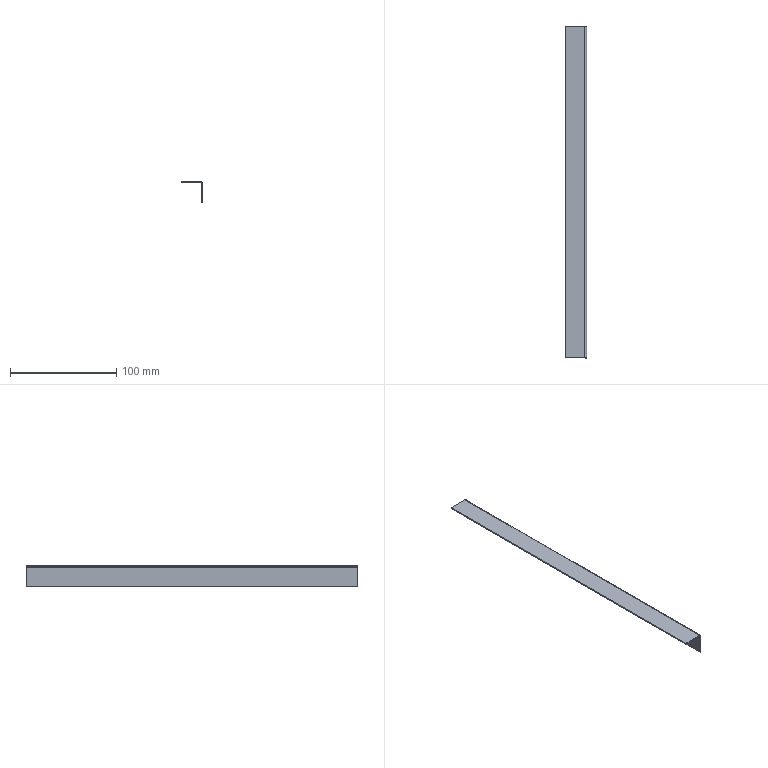Component | SolidWorks | CCQ-1.1-22VerticalAngleIron-1 | 1 solid | 14 faces | box 20 x 312 x 20 mm | volume 12002 mm3 | plane 12 | cylinder 2 | commonest cylinder face diameters 1.473 x1 3.473 x1 | material 304
STEP:
#1=COLOUR_RGB('',0.7922,0.8196,0.9333);
#2=FILL_AREA_STYLE_COLOUR('',#1);
#3=FILL_AREA_STYLE('',(#2));
#4=SURFACE_STYLE_FILL_AREA(#3);
#5=SURFACE_SIDE_STYLE('',(#4));
#6=SURFACE_STYLE_USAGE(.BOTH.,#5);
#7=PRESENTATION_STYLE_ASSIGNMENT((#6));
#8=CARTESIAN_POINT('',(0.6009,-4.902,-7.953));
#9=VERTEX_POINT('',#8);
#10=CARTESIAN_POINT('',(0.6009,-4.902,-7.992));
#11=VERTEX_POINT('',#10);
#12=CARTESIAN_POINT('',(0.6009,-4.902,-7.953));
#13=DIRECTION('',(-0.,0.,-1.));
#14=VECTOR('',#13,39.37);
#15=LINE('',#12,#14);
#16=EDGE_CURVE('',#9,#11,#15,.T.);
#17=ORIENTED_EDGE('',*,*,#16,.F.);
#18=CARTESIAN_POINT('',(0.6693,-4.902,-8.021));
#19=VERTEX_POINT('',#18);
#20=CARTESIAN_POINT('',(0.6009,-4.902,-8.021));
#21=DIRECTION('',(-0.,1.,0.));
#22=DIRECTION('',(0.,0.,1.));
#23=AXIS2_PLACEMENT_3D('',#20,#21,#22);
#24=CIRCLE('',#23,0.06837);
#25=EDGE_CURVE('',#9,#19,#24,.T.);
#26=ORIENTED_EDGE('',*,*,#25,.T.);
#27=CARTESIAN_POINT('',(0.6299,-4.902,-8.021));
#28=VERTEX_POINT('',#27);
#29=CARTESIAN_POINT('',(0.6299,-4.902,-8.021));
#30=DIRECTION('',(1.,0.,0.));
#31=VECTOR('',#30,39.37);
#32=LINE('',#29,#31);
#33=EDGE_CURVE('',#28,#19,#32,.T.);
#34=ORIENTED_EDGE('',*,*,#33,.F.);
#35=CARTESIAN_POINT('',(0.6009,-4.902,-8.021));
#36=DIRECTION('',(-0.,1.,0.));
#37=DIRECTION('',(-0.,0.,-1.));
#38=AXIS2_PLACEMENT_3D('',#35,#36,#37);
#39=CIRCLE('',#38,0.029);
#40=EDGE_CURVE('',#11,#28,#39,.T.);
#41=ORIENTED_EDGE('',*,*,#40,.F.);
#42=EDGE_LOOP('',(#17,#26,#34,#41));
#43=FACE_OUTER_BOUND('',#42,.T.);
#44=CARTESIAN_POINT('',(0.6009,-4.902,-7.953));
#45=DIRECTION('',(-0.,1.,0.));
#46=DIRECTION('',(-0.,0.,-1.));
#47=AXIS2_PLACEMENT_3D('',#44,#45,#46);
#48=PLANE('',#47);
#49=ADVANCED_FACE('',(#43),#48,.T.);
#50=CARTESIAN_POINT('',(-0.1181,-4.902,-7.953));
#51=VERTEX_POINT('',#50);
#52=CARTESIAN_POINT('',(-0.1181,-4.902,-7.953));
#53=DIRECTION('',(1.,0.,0.));
#54=VECTOR('',#53,39.37);
#55=LINE('',#52,#54);
#56=EDGE_CURVE('',#51,#9,#55,.T.);
#57=ORIENTED_EDGE('',*,*,#56,.T.);
#58=ORIENTED_EDGE('',*,*,#16,.T.);
#59=CARTESIAN_POINT('',(-0.1181,-4.902,-7.992));
#60=VERTEX_POINT('',#59);
#61=CARTESIAN_POINT('',(-0.1181,-4.902,-7.992));
#62=DIRECTION('',(1.,0.,0.));
#63=VECTOR('',#62,39.37);
#64=LINE('',#61,#63);
#65=EDGE_CURVE('',#60,#11,#64,.T.);
#66=ORIENTED_EDGE('',*,*,#65,.F.);
#67=CARTESIAN_POINT('',(-0.1181,-4.902,-7.953));
#68=DIRECTION('',(-0.,0.,-1.));
#69=VECTOR('',#68,39.37);
#70=LINE('',#67,#69);
#71=EDGE_CURVE('',#51,#60,#70,.T.);
#72=ORIENTED_EDGE('',*,*,#71,.F.);
#73=EDGE_LOOP('',(#57,#58,#66,#72));
#74=FACE_OUTER_BOUND('',#73,.T.);
#75=CARTESIAN_POINT('',(0.6299,-4.902,-8.021));
#76=DIRECTION('',(-0.,1.,0.));
#77=DIRECTION('',(-0.,0.,-1.));
#78=AXIS2_PLACEMENT_3D('',#75,#76,#77);
#79=PLANE('',#78);
#80=ADVANCED_FACE('',(#74),#79,.T.);
#81=CARTESIAN_POINT('',(0.6693,-17.185,-8.021));
#82=VERTEX_POINT('',#81);
#83=CARTESIAN_POINT('',(0.6299,-17.185,-8.021));
#84=VERTEX_POINT('',#83);
#85=CARTESIAN_POINT('',(0.6693,-17.185,-8.021));
#86=DIRECTION('',(-1.,-0.,-0.));
#87=VECTOR('',#86,39.37);
#88=LINE('',#85,#87);
#89=EDGE_CURVE('',#82,#84,#88,.T.);
#90=ORIENTED_EDGE('',*,*,#89,.F.);
#91=CARTESIAN_POINT('',(0.6009,-17.185,-7.953));
#92=VERTEX_POINT('',#91);
#93=CARTESIAN_POINT('',(0.6009,-17.185,-8.021));
#94=DIRECTION('',(-0.,1.,0.));
#95=DIRECTION('',(0.,0.,1.));
#96=AXIS2_PLACEMENT_3D('',#93,#94,#95);
#97=CIRCLE('',#96,0.06837);
#98=EDGE_CURVE('',#92,#82,#97,.T.);
#99=ORIENTED_EDGE('',*,*,#98,.F.);
#100=CARTESIAN_POINT('',(0.6009,-17.185,-7.992));
#101=VERTEX_POINT('',#100);
#102=CARTESIAN_POINT('',(0.6009,-17.185,-7.992));
#103=DIRECTION('',(0.,-0.,1.));
#104=VECTOR('',#103,39.37);
#105=LINE('',#102,#104);
#106=EDGE_CURVE('',#101,#92,#105,.T.);
#107=ORIENTED_EDGE('',*,*,#106,.F.);
#108=CARTESIAN_POINT('',(0.6009,-17.185,-8.021));
#109=DIRECTION('',(-0.,1.,0.));
#110=DIRECTION('',(-0.,0.,-1.));
#111=AXIS2_PLACEMENT_3D('',#108,#109,#110);
#112=CIRCLE('',#111,0.029);
#113=EDGE_CURVE('',#101,#84,#112,.T.);
#114=ORIENTED_EDGE('',*,*,#113,.T.);
#115=EDGE_LOOP('',(#90,#99,#107,#114));
#116=FACE_OUTER_BOUND('',#115,.T.);
#117=CARTESIAN_POINT('',(0.6693,-17.185,-8.021));
#118=DIRECTION('',(0.,-1.,-0.));
#119=DIRECTION('',(0.,-0.,1.));
#120=AXIS2_PLACEMENT_3D('',#117,#118,#119);
#121=PLANE('',#120);
#122=ADVANCED_FACE('',(#116),#121,.T.);
#123=CARTESIAN_POINT('',(0.6693,-17.185,-8.74));
#124=VERTEX_POINT('',#123);
#125=CARTESIAN_POINT('',(0.6693,-17.185,-7.953));
#126=DIRECTION('',(-0.,0.,-1.));
#127=VECTOR('',#126,39.37);
#128=LINE('',#125,#127);
#129=EDGE_CURVE('',#82,#124,#128,.T.);
#130=ORIENTED_EDGE('',*,*,#129,.F.);
#131=ORIENTED_EDGE('',*,*,#89,.T.);
#132=CARTESIAN_POINT('',(0.6299,-17.185,-8.74));
#133=VERTEX_POINT('',#132);
#134=CARTESIAN_POINT('',(0.6299,-17.185,-7.953));
#135=DIRECTION('',(-0.,0.,-1.));
#136=VECTOR('',#135,39.37);
#137=LINE('',#134,#136);
#138=EDGE_CURVE('',#84,#133,#137,.T.);
#139=ORIENTED_EDGE('',*,*,#138,.T.);
#140=CARTESIAN_POINT('',(0.6299,-17.185,-8.74));
#141=DIRECTION('',(1.,0.,0.));
#142=VECTOR('',#141,39.37);
#143=LINE('',#140,#142);
#144=EDGE_CURVE('',#133,#124,#143,.T.);
#145=ORIENTED_EDGE('',*,*,#144,.T.);
#146=EDGE_LOOP('',(#130,#131,#139,#145));
#147=FACE_OUTER_BOUND('',#146,.T.);
#148=CARTESIAN_POINT('',(0.6009,-17.185,-7.992));
#149=DIRECTION('',(0.,-1.,-0.));
#150=DIRECTION('',(0.,-0.,1.));
#151=AXIS2_PLACEMENT_3D('',#148,#149,#150);
#152=PLANE('',#151);
#153=ADVANCED_FACE('',(#147),#152,.T.);
#154=ORIENTED_EDGE('',*,*,#129,.T.);
#155=CARTESIAN_POINT('',(0.6693,-4.902,-8.74));
#156=VERTEX_POINT('',#155);
#157=CARTESIAN_POINT('',(0.6693,-4.902,-8.74));
#158=DIRECTION('',(0.,-1.,-0.));
#159=VECTOR('',#158,39.37);
#160=LINE('',#157,#159);
#161=EDGE_CURVE('',#156,#124,#160,.T.);
#162=ORIENTED_EDGE('',*,*,#161,.F.);
#163=CARTESIAN_POINT('',(0.6693,-4.902,-7.953));
#164=DIRECTION('',(-0.,0.,-1.));
#165=VECTOR('',#164,39.37);
#166=LINE('',#163,#165);
#167=EDGE_CURVE('',#19,#156,#166,.T.);
#168=ORIENTED_EDGE('',*,*,#167,.F.);
#169=CARTESIAN_POINT('',(0.6693,-4.902,-8.021));
#170=DIRECTION('',(0.,-1.,-0.));
#171=VECTOR('',#170,39.37);
#172=LINE('',#169,#171);
#173=EDGE_CURVE('',#19,#82,#172,.T.);
#174=ORIENTED_EDGE('',*,*,#173,.T.);
#175=EDGE_LOOP('',(#154,#162,#168,#174));
#176=FACE_OUTER_BOUND('',#175,.T.);
#177=CARTESIAN_POINT('',(0.6693,-4.902,-7.953));
#178=DIRECTION('',(-1.,-0.,-0.));
#179=DIRECTION('',(-0.,1.,0.));
#180=AXIS2_PLACEMENT_3D('',#177,#178,#179);
#181=PLANE('',#180);
#182=ADVANCED_FACE('',(#176),#181,.F.);
#183=ORIENTED_EDGE('',*,*,#144,.F.);
#184=CARTESIAN_POINT('',(0.6299,-4.902,-8.74));
#185=VERTEX_POINT('',#184);
#186=CARTESIAN_POINT('',(0.6299,-4.902,-8.74));
#187=DIRECTION('',(0.,-1.,-0.));
#188=VECTOR('',#187,39.37);
#189=LINE('',#186,#188);
#190=EDGE_CURVE('',#185,#133,#189,.T.);
#191=ORIENTED_EDGE('',*,*,#190,.F.);
#192=CARTESIAN_POINT('',(0.6299,-4.902,-8.74));
#193=DIRECTION('',(1.,0.,0.));
#194=VECTOR('',#193,39.37);
#195=LINE('',#192,#194);
#196=EDGE_CURVE('',#185,#156,#195,.T.);
#197=ORIENTED_EDGE('',*,*,#196,.T.);
#198=ORIENTED_EDGE('',*,*,#161,.T.);
#199=EDGE_LOOP('',(#183,#191,#197,#198));
#200=FACE_OUTER_BOUND('',#199,.T.);
#201=CARTESIAN_POINT('',(0.6299,-4.902,-8.74));
#202=DIRECTION('',(-0.,0.,-1.));
#203=DIRECTION('',(0.,-1.,-0.));
#204=AXIS2_PLACEMENT_3D('',#201,#202,#203);
#205=PLANE('',#204);
#206=ADVANCED_FACE('',(#200),#205,.T.);
#207=ORIENTED_EDGE('',*,*,#138,.F.);
#208=CARTESIAN_POINT('',(0.6299,-4.902,-8.021));
#209=DIRECTION('',(0.,-1.,-0.));
#210=VECTOR('',#209,39.37);
#211=LINE('',#208,#210);
#212=EDGE_CURVE('',#28,#84,#211,.T.);
#213=ORIENTED_EDGE('',*,*,#212,.F.);
#214=CARTESIAN_POINT('',(0.6299,-4.902,-7.953));
#215=DIRECTION('',(-0.,0.,-1.));
#216=VECTOR('',#215,39.37);
#217=LINE('',#214,#216);
#218=EDGE_CURVE('',#28,#185,#217,.T.);
#219=ORIENTED_EDGE('',*,*,#218,.T.);
#220=ORIENTED_EDGE('',*,*,#190,.T.);
#221=EDGE_LOOP('',(#207,#213,#219,#220));
#222=FACE_OUTER_BOUND('',#221,.T.);
#223=CARTESIAN_POINT('',(0.6299,-4.902,-7.953));
#224=DIRECTION('',(-1.,-0.,-0.));
#225=DIRECTION('',(-0.,1.,0.));
#226=AXIS2_PLACEMENT_3D('',#223,#224,#225);
#227=PLANE('',#226);
#228=ADVANCED_FACE('',(#222),#227,.T.);
#229=ORIENTED_EDGE('',*,*,#113,.F.);
#230=CARTESIAN_POINT('',(0.6009,-4.902,-7.992));
#231=DIRECTION('',(0.,-1.,-0.));
#232=VECTOR('',#231,39.37);
#233=LINE('',#230,#232);
#234=EDGE_CURVE('',#11,#101,#233,.T.);
#235=ORIENTED_EDGE('',*,*,#234,.F.);
#236=ORIENTED_EDGE('',*,*,#40,.T.);
#237=ORIENTED_EDGE('',*,*,#212,.T.);
#238=EDGE_LOOP('',(#229,#235,#236,#237));
#239=FACE_OUTER_BOUND('',#238,.T.);
#240=CARTESIAN_POINT('',(0.6009,-4.902,-8.021));
#241=DIRECTION('',(0.,-1.,-0.));
#242=DIRECTION('',(0.,0.,1.));
#243=AXIS2_PLACEMENT_3D('',#240,#241,#242);
#244=CYLINDRICAL_SURFACE('',#243,0.029);
#245=ADVANCED_FACE('',(#239),#244,.F.);
#246=CARTESIAN_POINT('',(-0.1181,-17.185,-7.992));
#247=VERTEX_POINT('',#246);
#248=CARTESIAN_POINT('',(-0.1181,-17.185,-7.992));
#249=DIRECTION('',(1.,0.,0.));
#250=VECTOR('',#249,39.37);
#251=LINE('',#248,#250);
#252=EDGE_CURVE('',#247,#101,#251,.T.);
#253=ORIENTED_EDGE('',*,*,#252,.F.);
#254=CARTESIAN_POINT('',(-0.1181,-4.902,-7.992));
#255=DIRECTION('',(0.,-1.,-0.));
#256=VECTOR('',#255,39.37);
#257=LINE('',#254,#256);
#258=EDGE_CURVE('',#60,#247,#257,.T.);
#259=ORIENTED_EDGE('',*,*,#258,.F.);
#260=ORIENTED_EDGE('',*,*,#65,.T.);
#261=ORIENTED_EDGE('',*,*,#234,.T.);
#262=EDGE_LOOP('',(#253,#259,#260,#261));
#263=FACE_OUTER_BOUND('',#262,.T.);
#264=CARTESIAN_POINT('',(-0.1181,-4.902,-7.992));
#265=DIRECTION('',(-0.,0.,-1.));
#266=DIRECTION('',(0.,-1.,-0.));
#267=AXIS2_PLACEMENT_3D('',#264,#265,#266);
#268=PLANE('',#267);
#269=ADVANCED_FACE('',(#263),#268,.T.);
#270=CARTESIAN_POINT('',(-0.1181,-17.185,-7.953));
#271=VERTEX_POINT('',#270);
#272=CARTESIAN_POINT('',(-0.1181,-17.185,-7.953));
#273=DIRECTION('',(-0.,0.,-1.));
#274=VECTOR('',#273,39.37);
#275=LINE('',#272,#274);
#276=EDGE_CURVE('',#271,#247,#275,.T.);
#277=ORIENTED_EDGE('',*,*,#276,.F.);
#278=CARTESIAN_POINT('',(-0.1181,-4.902,-7.953));
#279=DIRECTION('',(0.,-1.,-0.));
#280=VECTOR('',#279,39.37);
#281=LINE('',#278,#280);
#282=EDGE_CURVE('',#51,#271,#281,.T.);
#283=ORIENTED_EDGE('',*,*,#282,.F.);
#284=ORIENTED_EDGE('',*,*,#71,.T.);
#285=ORIENTED_EDGE('',*,*,#258,.T.);
#286=EDGE_LOOP('',(#277,#283,#284,#285));
#287=FACE_OUTER_BOUND('',#286,.T.);
#288=CARTESIAN_POINT('',(-0.1181,-4.902,-7.953));
#289=DIRECTION('',(-1.,-0.,-0.));
#290=DIRECTION('',(-0.,1.,0.));
#291=AXIS2_PLACEMENT_3D('',#288,#289,#290);
#292=PLANE('',#291);
#293=ADVANCED_FACE('',(#287),#292,.T.);
#294=CARTESIAN_POINT('',(-0.1181,-17.185,-7.953));
#295=DIRECTION('',(1.,0.,0.));
#296=VECTOR('',#295,39.37);
#297=LINE('',#294,#296);
#298=EDGE_CURVE('',#271,#92,#297,.T.);
#299=ORIENTED_EDGE('',*,*,#298,.T.);
#300=CARTESIAN_POINT('',(0.6009,-4.902,-7.953));
#301=DIRECTION('',(0.,-1.,-0.));
#302=VECTOR('',#301,39.37);
#303=LINE('',#300,#302);
#304=EDGE_CURVE('',#9,#92,#303,.T.);
#305=ORIENTED_EDGE('',*,*,#304,.F.);
#306=ORIENTED_EDGE('',*,*,#56,.F.);
#307=ORIENTED_EDGE('',*,*,#282,.T.);
#308=EDGE_LOOP('',(#299,#305,#306,#307));
#309=FACE_OUTER_BOUND('',#308,.T.);
#310=CARTESIAN_POINT('',(-0.1181,-4.902,-7.953));
#311=DIRECTION('',(-0.,0.,-1.));
#312=DIRECTION('',(0.,-1.,-0.));
#313=AXIS2_PLACEMENT_3D('',#310,#311,#312);
#314=PLANE('',#313);
#315=ADVANCED_FACE('',(#309),#314,.F.);
#316=ORIENTED_EDGE('',*,*,#98,.T.);
#317=ORIENTED_EDGE('',*,*,#173,.F.);
#318=ORIENTED_EDGE('',*,*,#25,.F.);
#319=ORIENTED_EDGE('',*,*,#304,.T.);
#320=EDGE_LOOP('',(#316,#317,#318,#319));
#321=FACE_OUTER_BOUND('',#320,.T.);
#322=CARTESIAN_POINT('',(0.6009,-4.902,-8.021));
#323=DIRECTION('',(0.,-1.,-0.));
#324=DIRECTION('',(0.,0.,1.));
#325=AXIS2_PLACEMENT_3D('',#322,#323,#324);
#326=CYLINDRICAL_SURFACE('',#325,0.06837);
#327=ADVANCED_FACE('',(#321),#326,.T.);
#328=ORIENTED_EDGE('',*,*,#167,.T.);
#329=ORIENTED_EDGE('',*,*,#196,.F.);
#330=ORIENTED_EDGE('',*,*,#218,.F.);
#331=ORIENTED_EDGE('',*,*,#33,.T.);
#332=EDGE_LOOP('',(#328,#329,#330,#331));
#333=FACE_OUTER_BOUND('',#332,.T.);
#334=CARTESIAN_POINT('',(0.6009,-4.902,-8.021));
#335=DIRECTION('',(-0.,1.,0.));
#336=DIRECTION('',(-0.,0.,-1.));
#337=AXIS2_PLACEMENT_3D('',#334,#335,#336);
#338=PLANE('',#337);
#339=ADVANCED_FACE('',(#333),#338,.T.);
#340=ORIENTED_EDGE('',*,*,#252,.T.);
#341=ORIENTED_EDGE('',*,*,#106,.T.);
#342=ORIENTED_EDGE('',*,*,#298,.F.);
#343=ORIENTED_EDGE('',*,*,#276,.T.);
#344=EDGE_LOOP('',(#340,#341,#342,#343));
#345=FACE_OUTER_BOUND('',#344,.T.);
#346=CARTESIAN_POINT('',(0.6009,-17.185,-8.021));
#347=DIRECTION('',(-0.,1.,0.));
#348=DIRECTION('',(-0.,0.,-1.));
#349=AXIS2_PLACEMENT_3D('',#346,#347,#348);
#350=PLANE('',#349);
#351=ADVANCED_FACE('',(#345),#350,.F.);
#352=CLOSED_SHELL('',(#49,#80,#122,#153,#182,#206,#228,#245,#269,#293,#315,#327,#339,#351));
#353=MANIFOLD_SOLID_BREP('',#352);
#354=STYLED_ITEM('',(#7),#353);
#355=PRESENTATION_LAYER_ASSIGNMENT('','',(#354));
#356=(LENGTH_UNIT()NAMED_UNIT(*)SI_UNIT($,.METRE.));
#357=LENGTH_MEASURE_WITH_UNIT(LENGTH_MEASURE(0.0254),#356);
#358=DIMENSIONAL_EXPONENTS(1.,0.,0.,0.,0.,0.,0.);
#359=(CONVERSION_BASED_UNIT('',#357)LENGTH_UNIT()NAMED_UNIT(#358));
#360=UNCERTAINTY_MEASURE_WITH_UNIT(LENGTH_MEASURE(0.00001),#359,'','');
#361=(NAMED_UNIT(*)PLANE_ANGLE_UNIT()SI_UNIT($,.RADIAN.));
#362=(NAMED_UNIT(*)SI_UNIT($,.STERADIAN.)SOLID_ANGLE_UNIT());
#363=(GEOMETRIC_REPRESENTATION_CONTEXT(3)GLOBAL_UNCERTAINTY_ASSIGNED_CONTEXT((#360))GLOBAL_UNIT_ASSIGNED_CONTEXT((#359,#361,#362))REPRESENTATION_CONTEXT('',''));
#364=MECHANICAL_DESIGN_GEOMETRIC_PRESENTATION_REPRESENTATION('',(#354),#363);
#365=CARTESIAN_POINT('',(0.,0.,0.));
#366=DIRECTION('',(0.,0.,1.));
#367=DIRECTION('',(1.,0.,0.));
#368=AXIS2_PLACEMENT_3D('',#365,#366,#367);
#369=(LENGTH_UNIT()NAMED_UNIT(*)SI_UNIT($,.METRE.));
#370=LENGTH_MEASURE_WITH_UNIT(LENGTH_MEASURE(0.0254),#369);
#371=DIMENSIONAL_EXPONENTS(1.,0.,0.,0.,0.,0.,0.);
#372=(CONVERSION_BASED_UNIT('',#370)LENGTH_UNIT()NAMED_UNIT(#371));
#373=UNCERTAINTY_MEASURE_WITH_UNIT(LENGTH_MEASURE(0.00001),#372,'','');
#374=(NAMED_UNIT(*)PLANE_ANGLE_UNIT()SI_UNIT($,.RADIAN.));
#375=(NAMED_UNIT(*)SI_UNIT($,.STERADIAN.)SOLID_ANGLE_UNIT());
#376=(GEOMETRIC_REPRESENTATION_CONTEXT(3)GLOBAL_UNCERTAINTY_ASSIGNED_CONTEXT((#373))GLOBAL_UNIT_ASSIGNED_CONTEXT((#372,#374,#375))REPRESENTATION_CONTEXT('',''));
#377=ADVANCED_BREP_SHAPE_REPRESENTATION('',(#353,#368),#376);